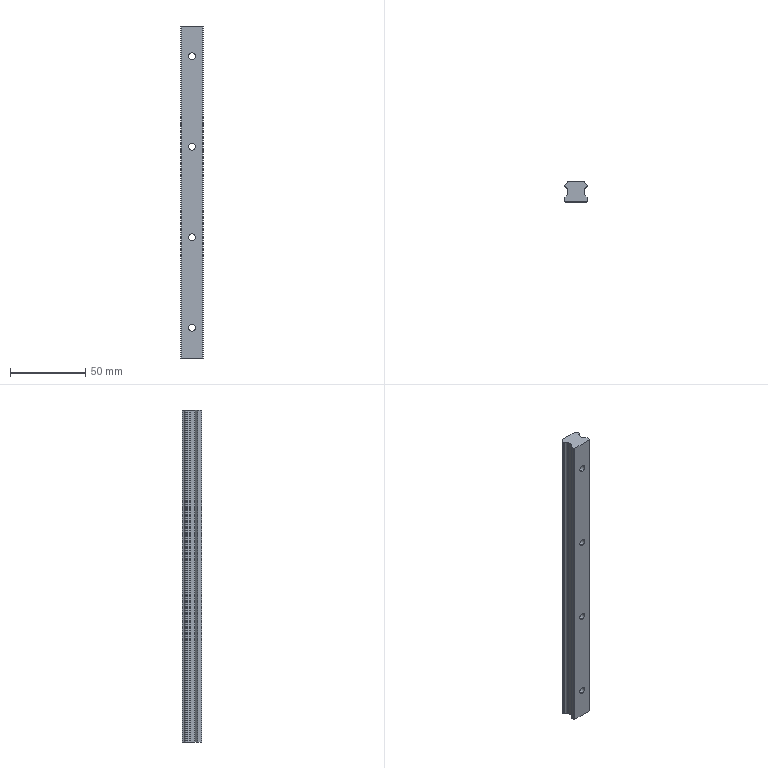Component | SolidWorks | F-YBCNS_1_1394078242-1_F-YBC_SHR28_220_r-1 | 1 solid | 58 faces | box 15 x 13 x 220 mm | volume 35417 mm3 | cylinder 34 | plane 24 | commonest cylinder face diameters 0.6 x14 4.5 x8 7.5 x8 2.862 x4
build123d program:
from build123d import *

# Parameters (mm, degrees)
BOSS_EXTRUDE1_DEPTH      = 110
BOSS_EXTRUDE1_DEPTH_BACK = 110


with BuildPart() as part:
    # Sketch1 → Boss-Extrude1 (new, two sides: drawn at the far end of the back side and taken through both)
    with BuildSketch(Plane.XY.offset(-BOSS_EXTRUDE1_DEPTH_BACK)):
        with BuildLine():
            Line((-7.5, 2.576), (-7.5, 0.5))
            Line((-7.5, 0.5), (-7, 0))
            Line((-7, 0), (7, 0))
            Line((7, 0), (7.5, 0.5))
            Line((7.5, 0.5), (7.5, 2.576))
            ThreePointArc((7.5, 2.576), (7.477, 2.691), (7.412, 2.788))
            Line((7.412, 2.788), (5.588, 4.612))
            ThreePointArc((5.588, 4.612), (5.523, 4.709), (5.5, 4.824))
            Line((5.5, 4.824), (5.5, 7.797))
            ThreePointArc((5.5, 7.797), (5.523, 7.912), (5.588, 8.009))
            Line((5.588, 8.009), (5.702, 8.123))
            ThreePointArc((5.702, 8.123), (5.763, 8.211), (5.789, 8.315))
            ThreePointArc((5.789, 8.315), (6.174, 9.2), (7.033, 9.64))
            ThreePointArc((7.033, 9.64), (7.171, 9.695), (7.266, 9.811))
            Line((7.266, 9.811), (7.5, 10.313))
            Line((7.5, 10.313), (7.5, 10.787))
            Line((7.5, 10.787), (7.265, 11.29))
            ThreePointArc((7.265, 11.29), (7.171, 11.406), (7.032, 11.461))
            ThreePointArc((7.032, 11.461), (6.192, 11.881), (5.794, 12.731))
            ThreePointArc((5.794, 12.731), (5.696, 12.923), (5.495, 13))
            Line((5.495, 13), (-5.495, 13))
            ThreePointArc((-5.495, 13), (-5.696, 12.923), (-5.794, 12.731))
            ThreePointArc((-5.794, 12.731), (-6.192, 11.881), (-7.032, 11.461))
            ThreePointArc((-7.032, 11.461), (-7.171, 11.406), (-7.265, 11.29))
            Line((-7.265, 11.29), (-7.5, 10.787))
            Line((-7.5, 10.787), (-7.5, 10.313))
            Line((-7.5, 10.313), (-7.266, 9.811))
            ThreePointArc((-7.266, 9.811), (-7.171, 9.695), (-7.033, 9.64))
            ThreePointArc((-7.033, 9.64), (-6.174, 9.2), (-5.789, 8.315))
            ThreePointArc((-5.789, 8.315), (-5.763, 8.211), (-5.702, 8.123))
            Line((-5.702, 8.123), (-5.588, 8.009))
            ThreePointArc((-5.588, 8.009), (-5.523, 7.912), (-5.5, 7.797))
            Line((-5.5, 7.797), (-5.5, 4.824))
            ThreePointArc((-5.5, 4.824), (-5.523, 4.709), (-5.588, 4.612))
            Line((-5.588, 4.612), (-7.412, 2.788))
            ThreePointArc((-7.412, 2.788), (-7.477, 2.691), (-7.5, 2.576))
        make_face()
    extrude(amount=BOSS_EXTRUDE1_DEPTH + BOSS_EXTRUDE1_DEPTH_BACK)

    # Sketch2 → Cut-Revolve1 (revolve, cut)
    with BuildSketch(Plane.XY.offset(90), mode=Mode.PRIVATE) as cut_revolve1_sk:
        Polygon((0, 13), (3.75, 13), (3.75, 7), (2.25, 7), (2.25, 0), (0, 0), align=None)
    revolve(cut_revolve1_sk.sketch.rotate(Axis((0, 0, 90), (0, 1, 0)), 270), axis=Axis((0, 0, 90), (0, 1, 0)), mode=Mode.SUBTRACT)

    # Sketch3 → Cut-Revolve2 (revolve, cut)
    with BuildSketch(Plane.XY.offset(-90), mode=Mode.PRIVATE) as cut_revolve2_sk:
        Polygon((0, 13), (3.75, 13), (3.75, 7), (2.25, 7), (2.25, 0), (0, 0), align=None)
    revolve(cut_revolve2_sk.sketch.rotate(Axis((0, 0, -90), (0, 1, 0)), 270), axis=Axis((0, 0, -90), (0, 1, 0)), mode=Mode.SUBTRACT)

    # Sketch4 → Cut-Revolve3 (revolve, cut)
    with BuildSketch(Plane.XY.offset(-30), mode=Mode.PRIVATE) as cut_revolve3_sk:
        Polygon((0, 13), (3.75, 13), (3.75, 7), (2.25, 7), (2.25, 0), (0, 0), align=None)
    revolve(cut_revolve3_sk.sketch.rotate(Axis((0, 0, -30), (0, 1, 0)), 270), axis=Axis((0, 0, -30), (0, 1, 0)), mode=Mode.SUBTRACT)

    # Sketch5 → Cut-Revolve4 (revolve, cut)
    with BuildSketch(Plane.XY.offset(30), mode=Mode.PRIVATE) as cut_revolve4_sk:
        Polygon((0, 13), (3.75, 13), (3.75, 7), (2.25, 7), (2.25, 0), (0, 0), align=None)
    revolve(cut_revolve4_sk.sketch.rotate(Axis((0, 0, 30), (0, 1, 0)), 270), axis=Axis((0, 0, 30), (0, 1, 0)), mode=Mode.SUBTRACT)


solid = part.part

# Placed as in the assembly
solid = solid.moved(Location((309.305, 292.175, 189.479), (0, 0, 0)))